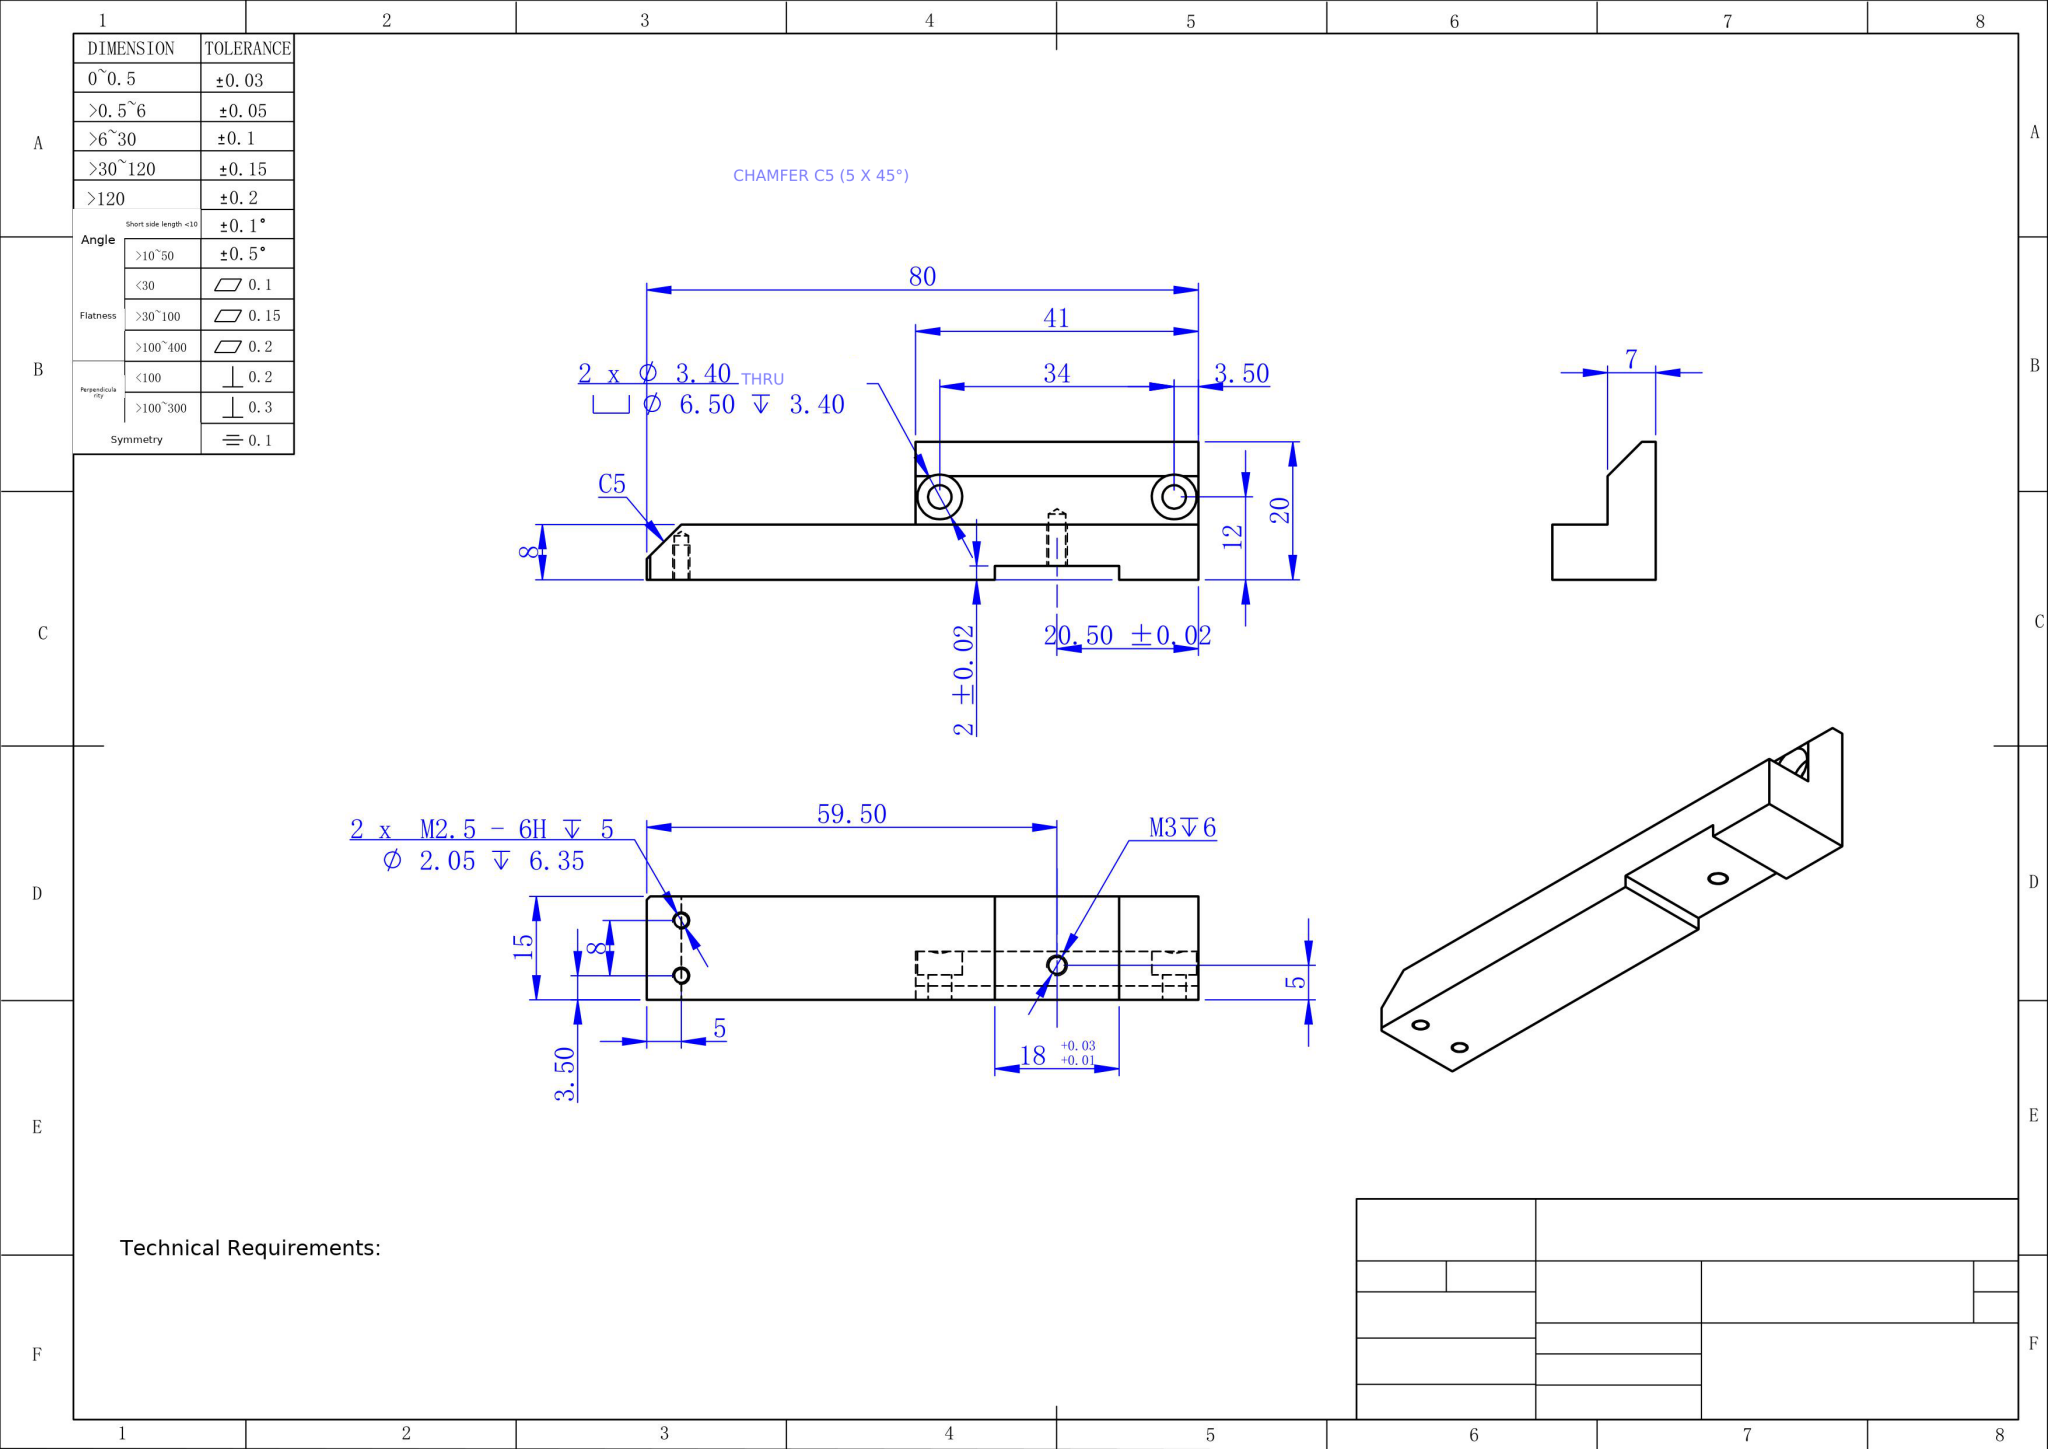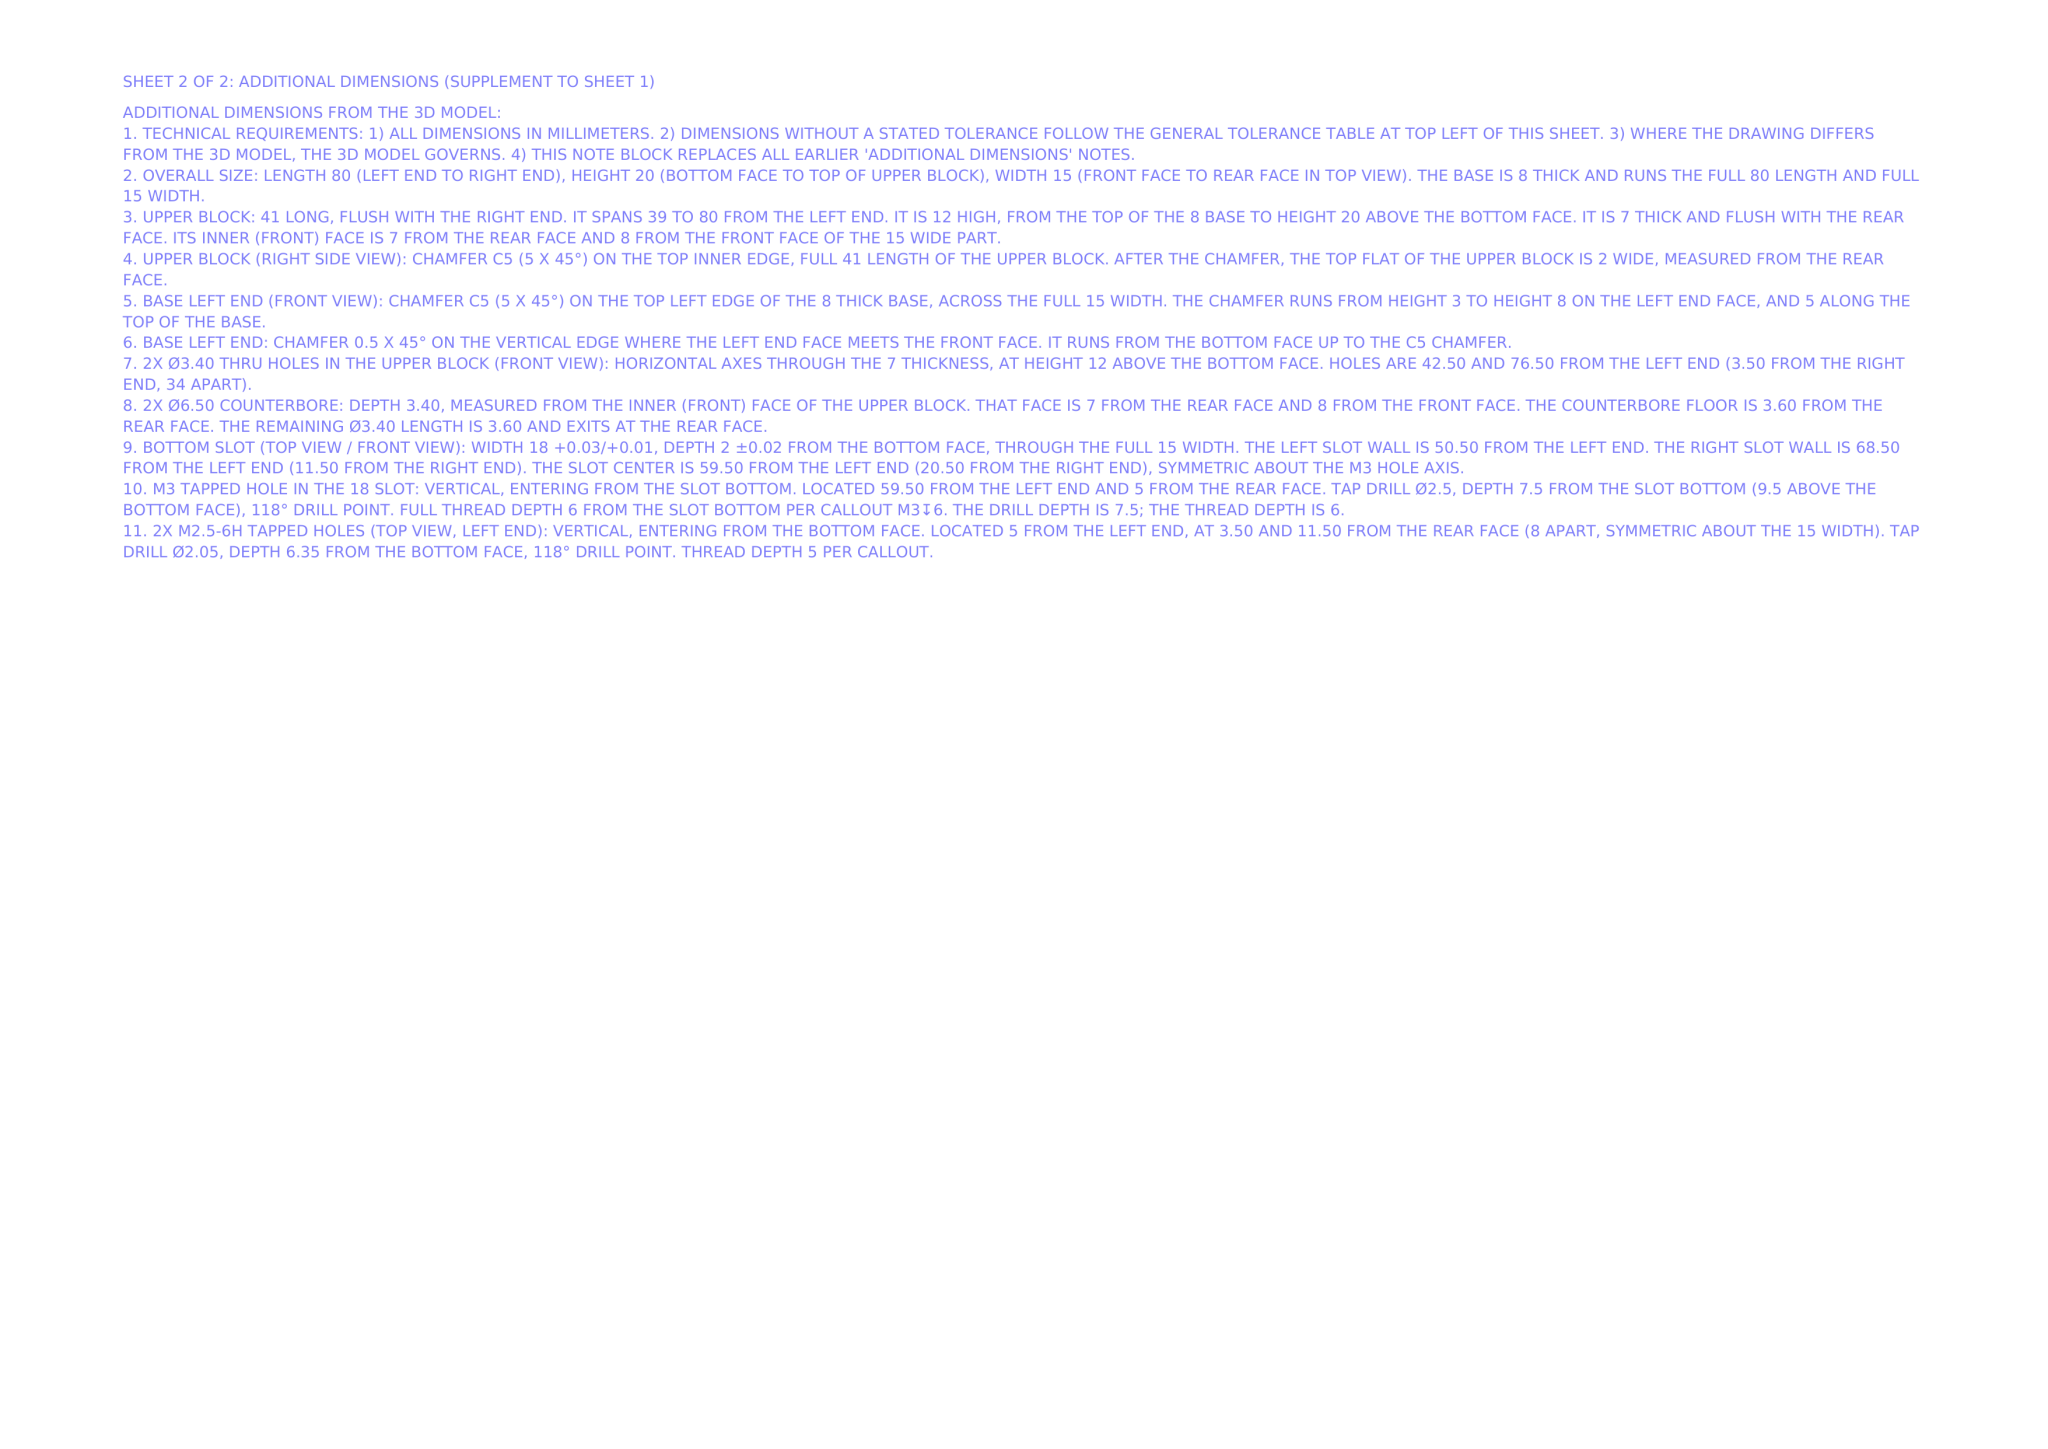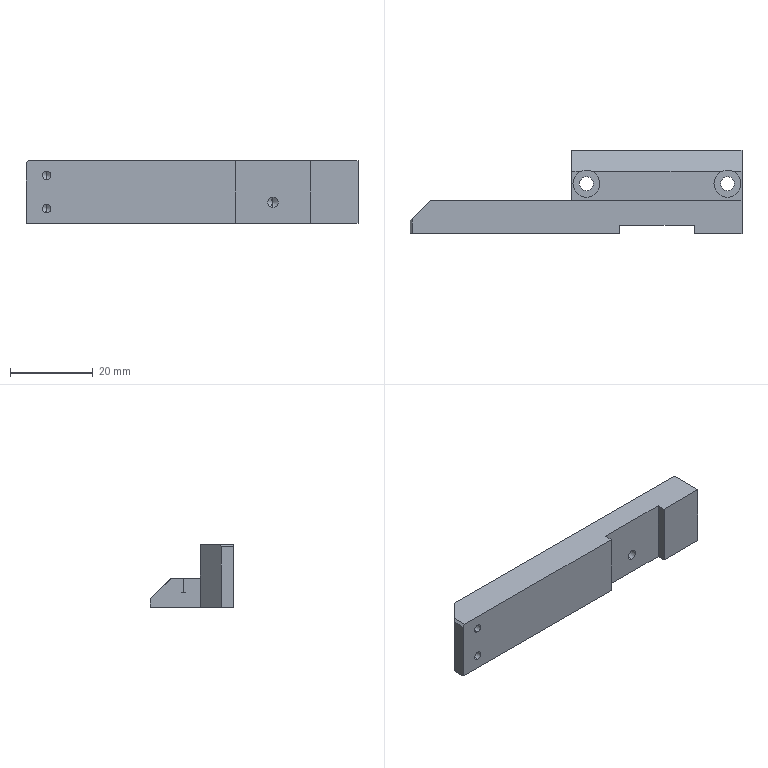Part | NX | mm | 1 solid | 38 faces | box 80 x 20 x 15 mm | volume 11431 mm3 | plane 18 | cylinder 14 | cone 6 | commonest cylinder face diameters 6.5 x4 3.4 x4 2.05 x4 2.5 x2